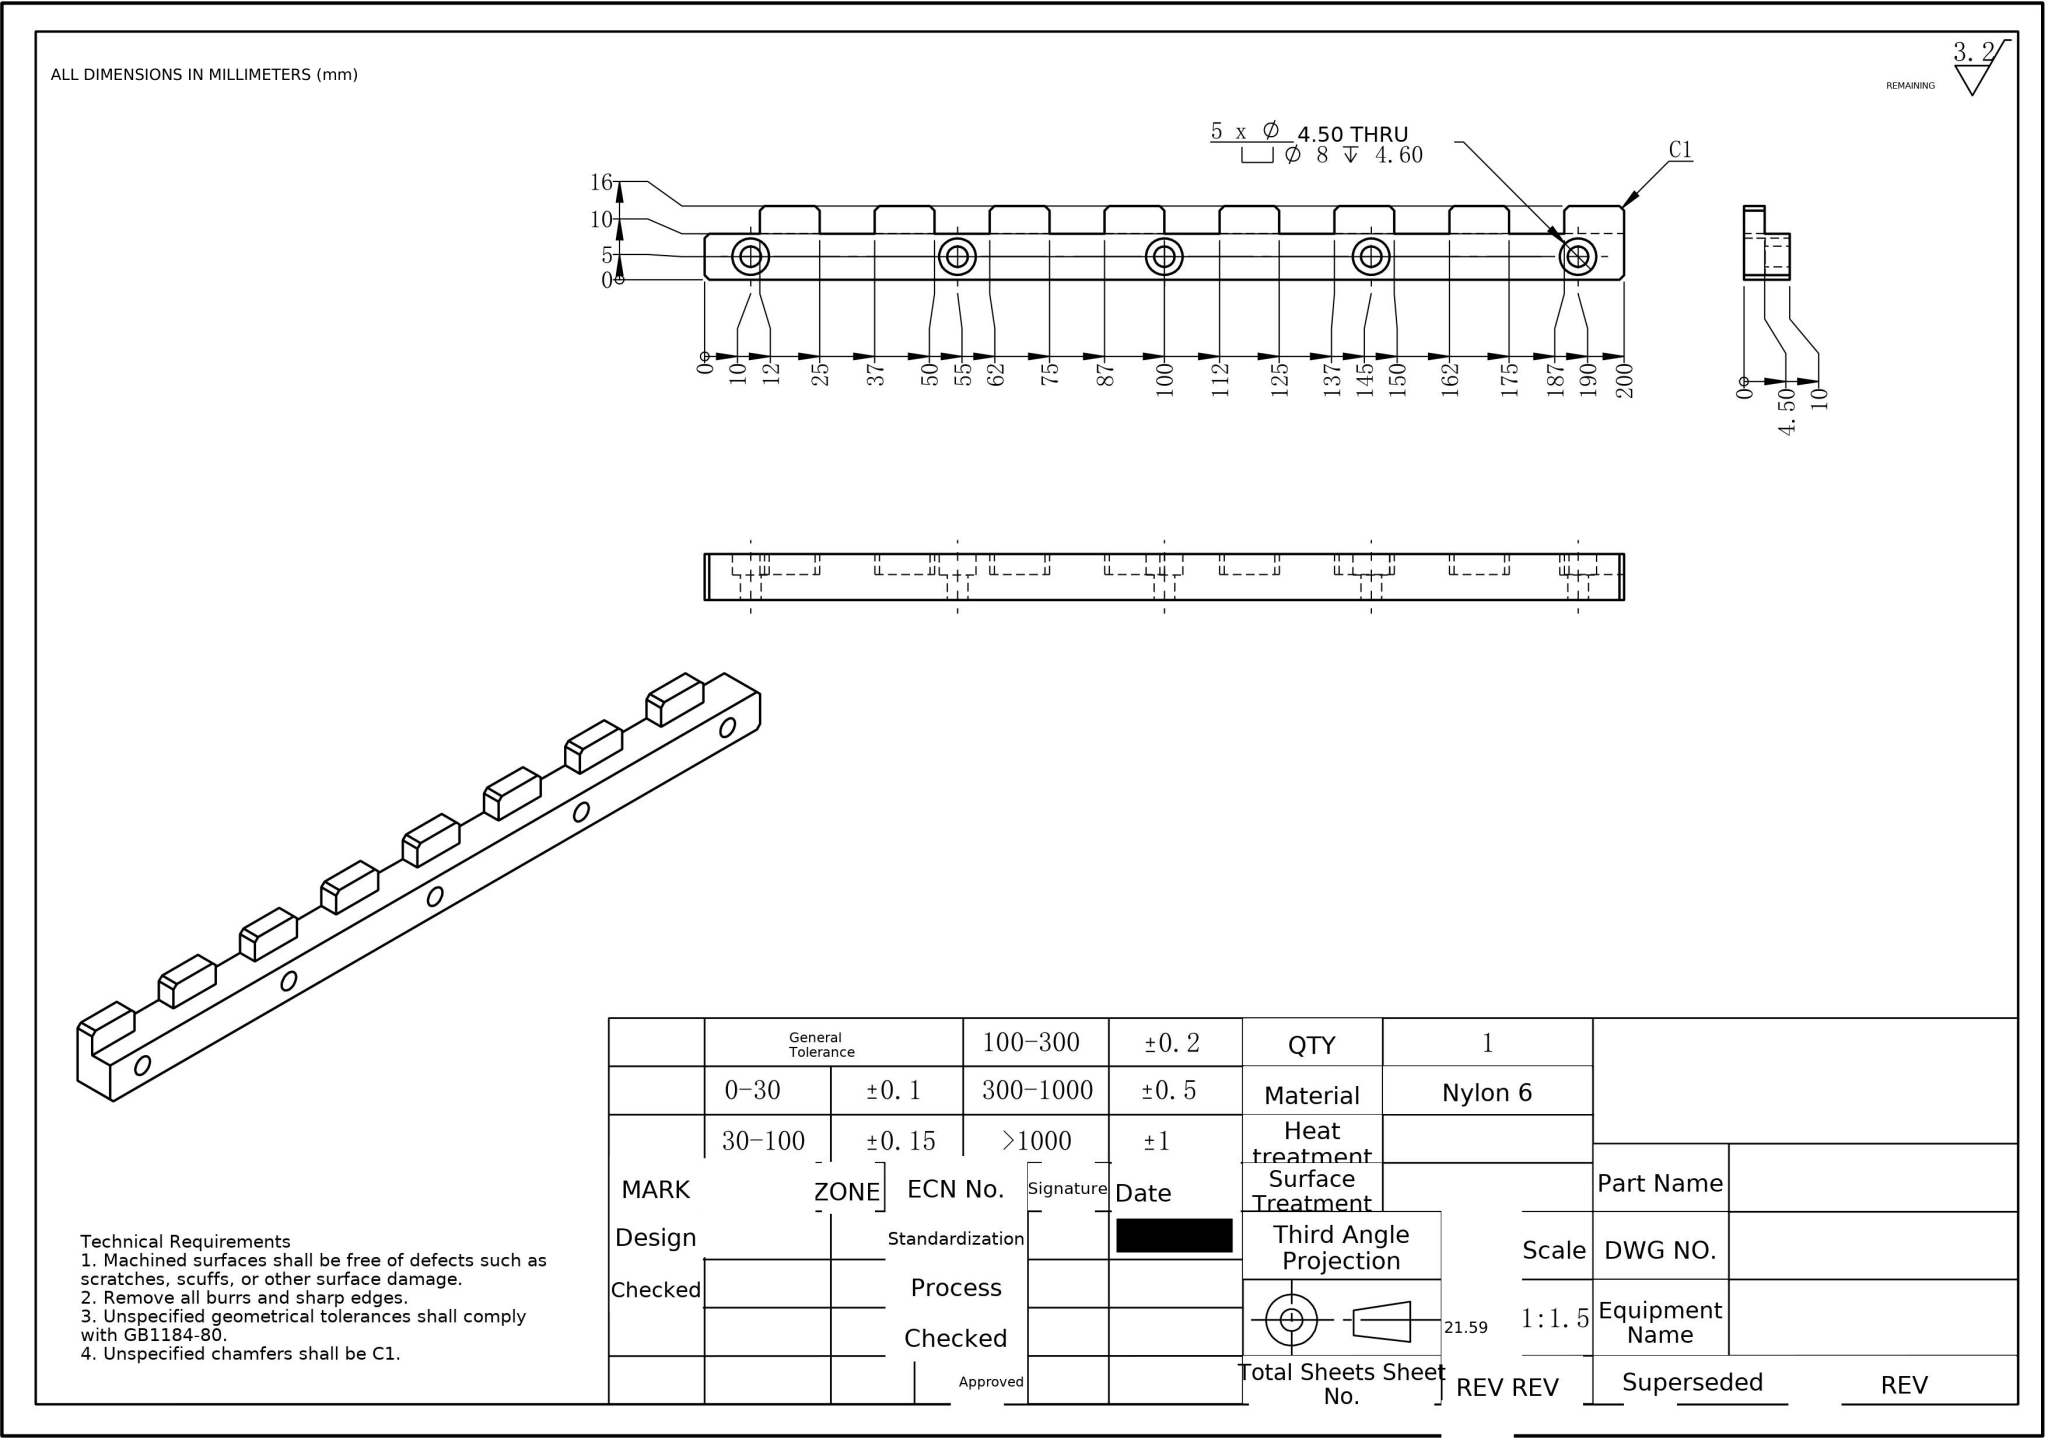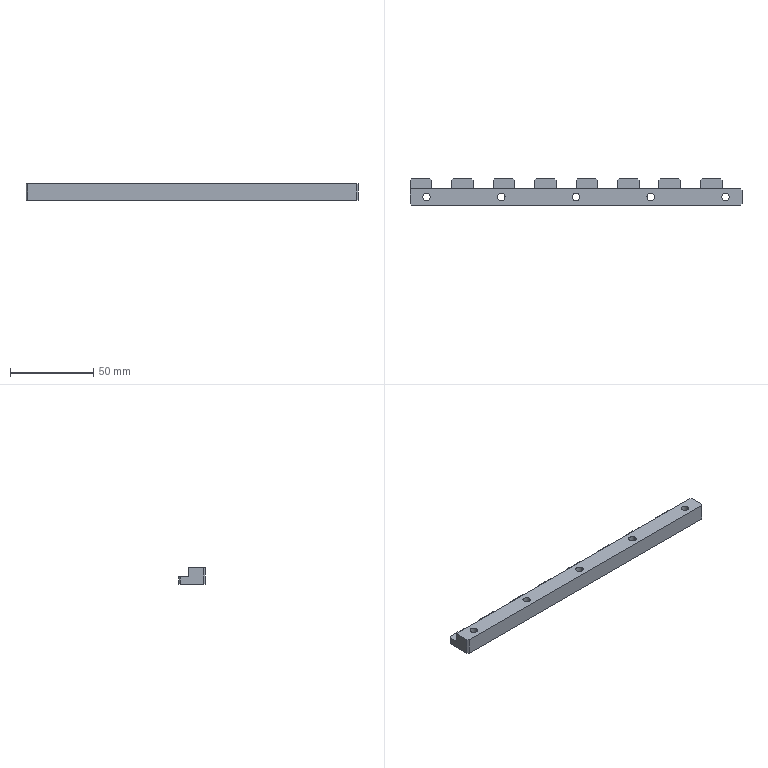Part | NX | mm | 1 solid | 81 faces | box 200 x 16 x 10 mm | volume 21171 mm3 | plane 61 | cylinder 20 | commonest cylinder face diameters 4.5 x10 8 x10